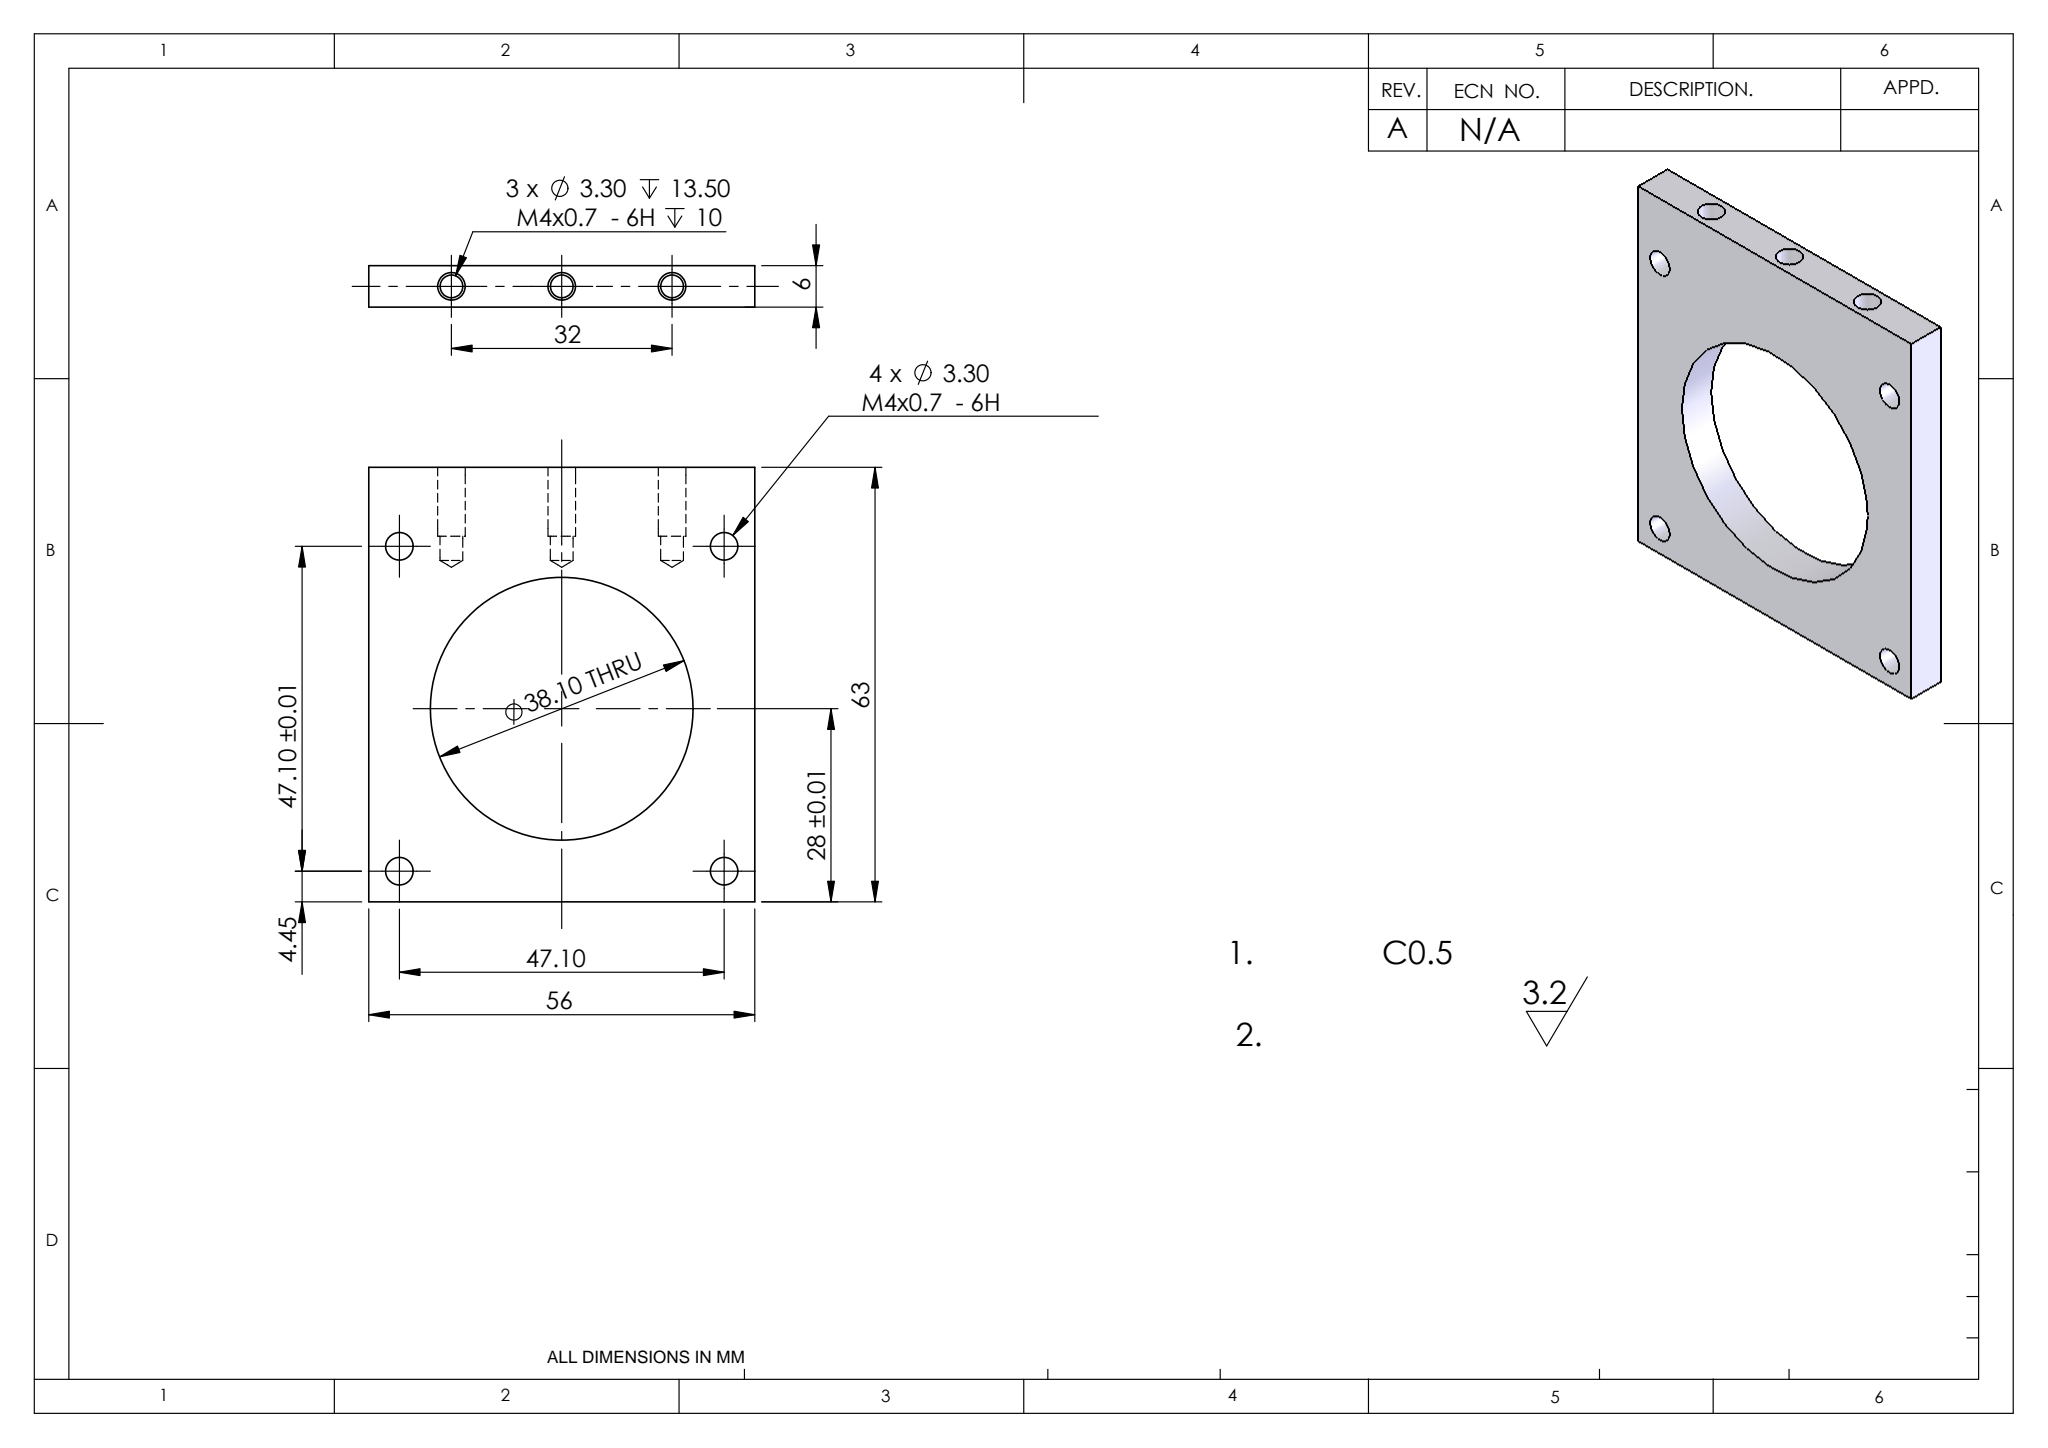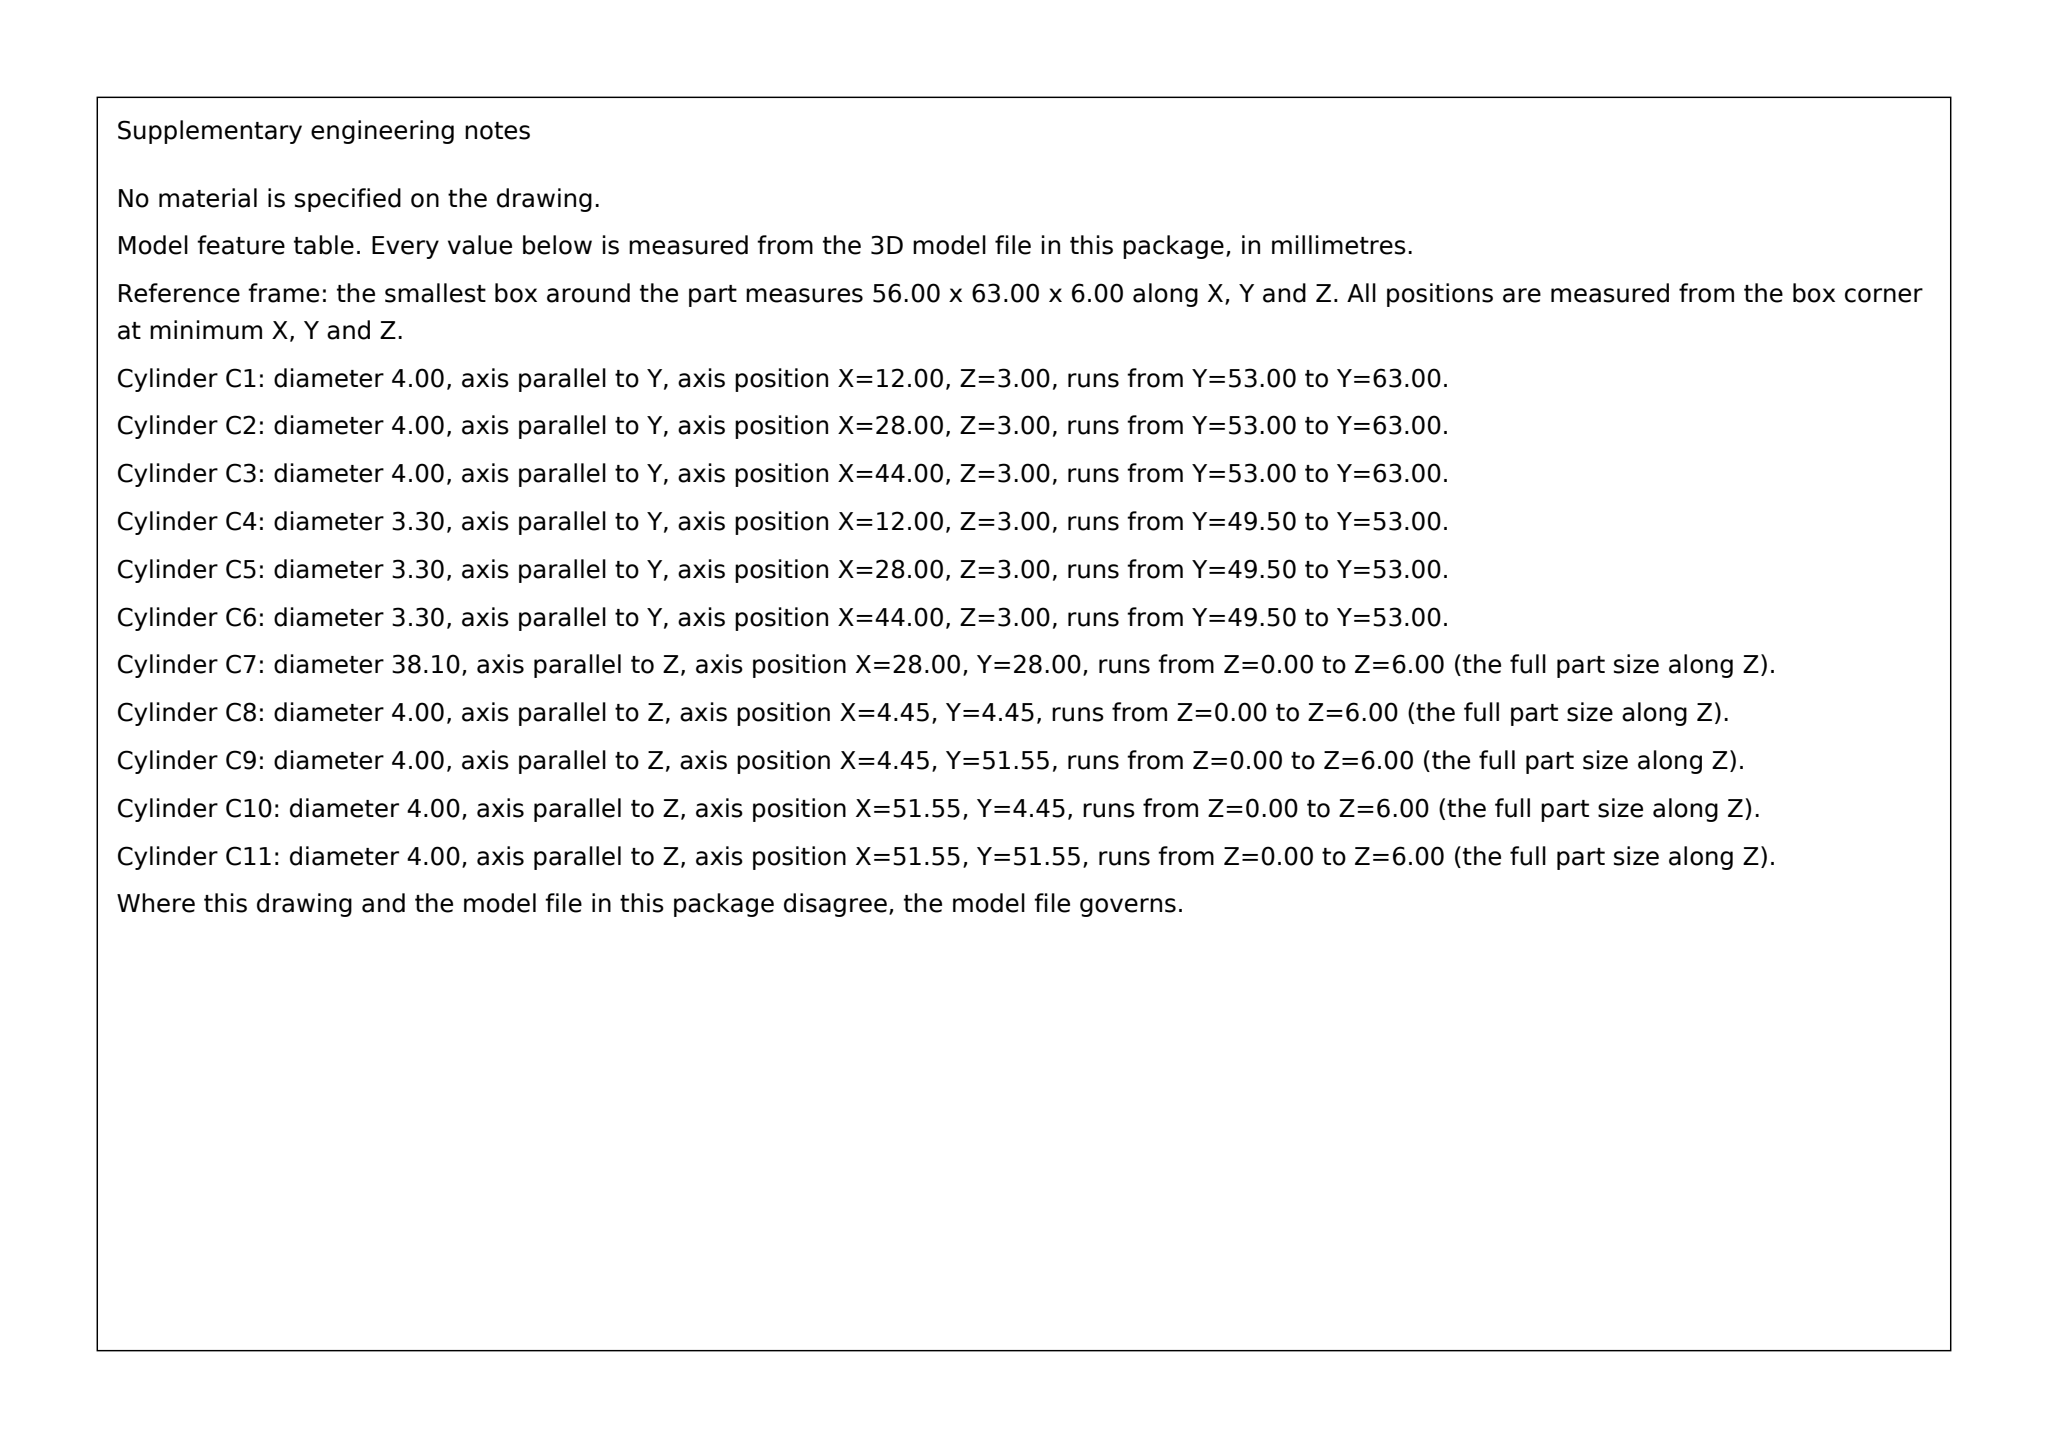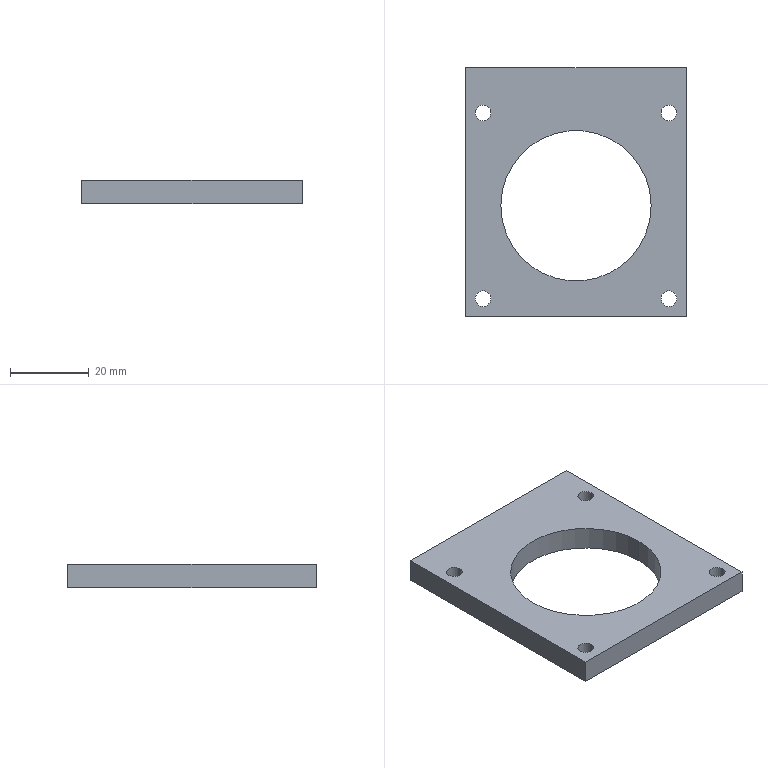Part | SolidWorks | mm | 1 solid | 37 faces | box 56 x 63 x 6 mm | volume 13551 mm3 | cylinder 22 | plane 9 | cone 6 | commonest cylinder face diameters 4 x14 3.3 x6 38.1 x2
build123d program:
from build123d import *

# Parameters (mm, degrees)
SKETCH1_W                   = 56
SKETCH1_H                   = 57
SKETCH1_R                   = 19.05
EXTRUDE1_DEPTH              = 6
M4_TAPPED_HOLE2_D           = 4
SKETCH5_W                   = 56
SKETCH5_H                   = 6
EXTRUDE2_DEPTH              = 6
M4_TAPPED_HOLE3_D           = 3.3
M4_TAPPED_HOLE3_DEPTH       = 13.5
M4_TAPPED_HOLE3_CBORE_D     = 4
M4_TAPPED_HOLE3_CBORE_DEPTH = 10
M4_TAPPED_HOLE3_TIP         = 0.9914


with BuildPart() as part:
    # Sketch1 → Extrude1 (new body)
    with BuildSketch(Plane.XY):
        with Locations((0, 0.5)):
            Rectangle(SKETCH1_W, SKETCH1_H)
        Circle(SKETCH1_R, mode=Mode.SUBTRACT)
    extrude(amount=EXTRUDE1_DEPTH)

    # M4 Tapped Hole2 (through all)
    with Locations(Plane(origin=(23.55, 23.55, 6), x_dir=(1, 0, 0), z_dir=(0, 0, 1))):
        with Locations((0, 0), (-47.1, 0), (-47.1, -47.1), (0, -47.1)):
            Hole(M4_TAPPED_HOLE2_D / 2)

    # Sketch5 → Extrude2 (add)
    with BuildSketch(Plane(origin=(0, 29, 0), x_dir=(-1, 0, 0), z_dir=(0, 1, 0))):
        with Locations((0, 3)):
            Rectangle(SKETCH5_W, SKETCH5_H)
    extrude(amount=EXTRUDE2_DEPTH)

    # M4 Tapped Hole3
    with Locations(Plane(origin=(16, 35, 3), x_dir=(0, 0, 1), z_dir=(0, 1, 0))):
        with Locations((0, 0), (0, -32), (0, -16)):
            CounterBoreHole(M4_TAPPED_HOLE3_D / 2, M4_TAPPED_HOLE3_CBORE_D / 2, M4_TAPPED_HOLE3_CBORE_DEPTH, depth=M4_TAPPED_HOLE3_DEPTH)
            with Locations((0, 0, -(M4_TAPPED_HOLE3_DEPTH + M4_TAPPED_HOLE3_TIP / 2))):  # 118° drill point
                Cone(0, M4_TAPPED_HOLE3_D / 2, M4_TAPPED_HOLE3_TIP, mode=Mode.SUBTRACT)


solid = part.part